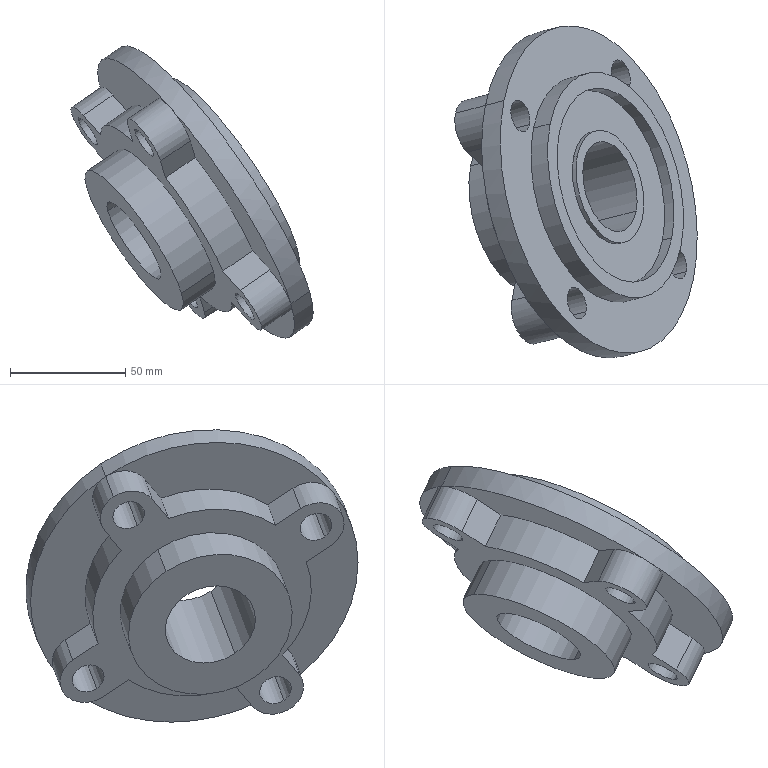Component | SolidWorks | UCFC208Bearing-1 | 1 solid | 47 faces | volume 356918 mm3 | cylinder 29 | plane 18 | commonest cylinder face diameters 14 x8 25 x5 96.828 x4 50 x2 86 x2 100 x2 145 x2 72.56 x2